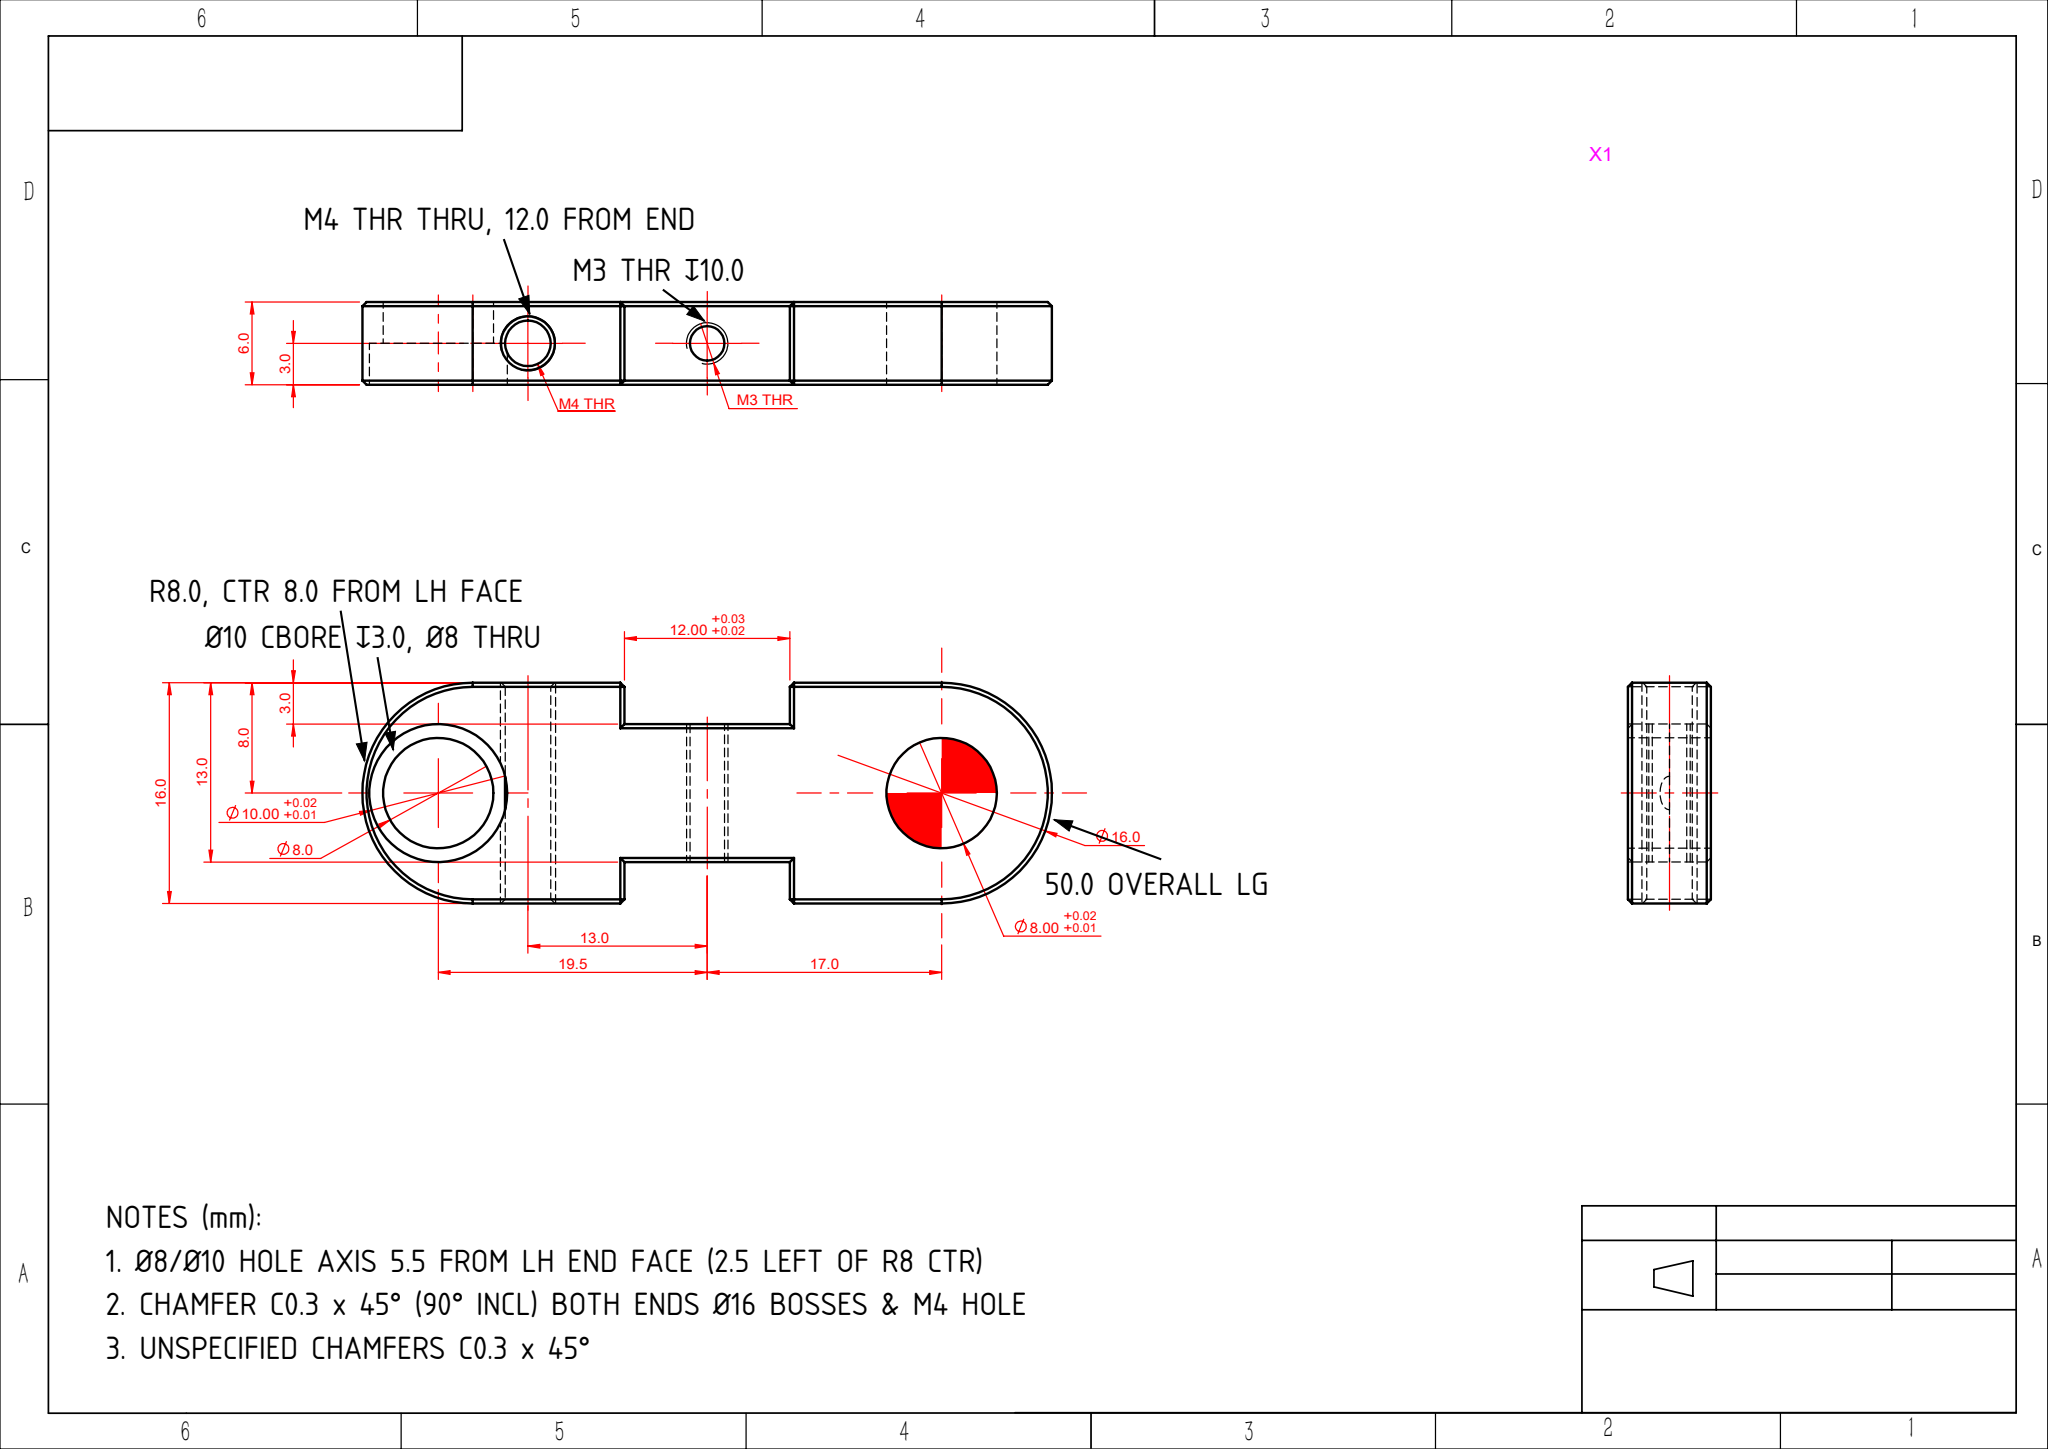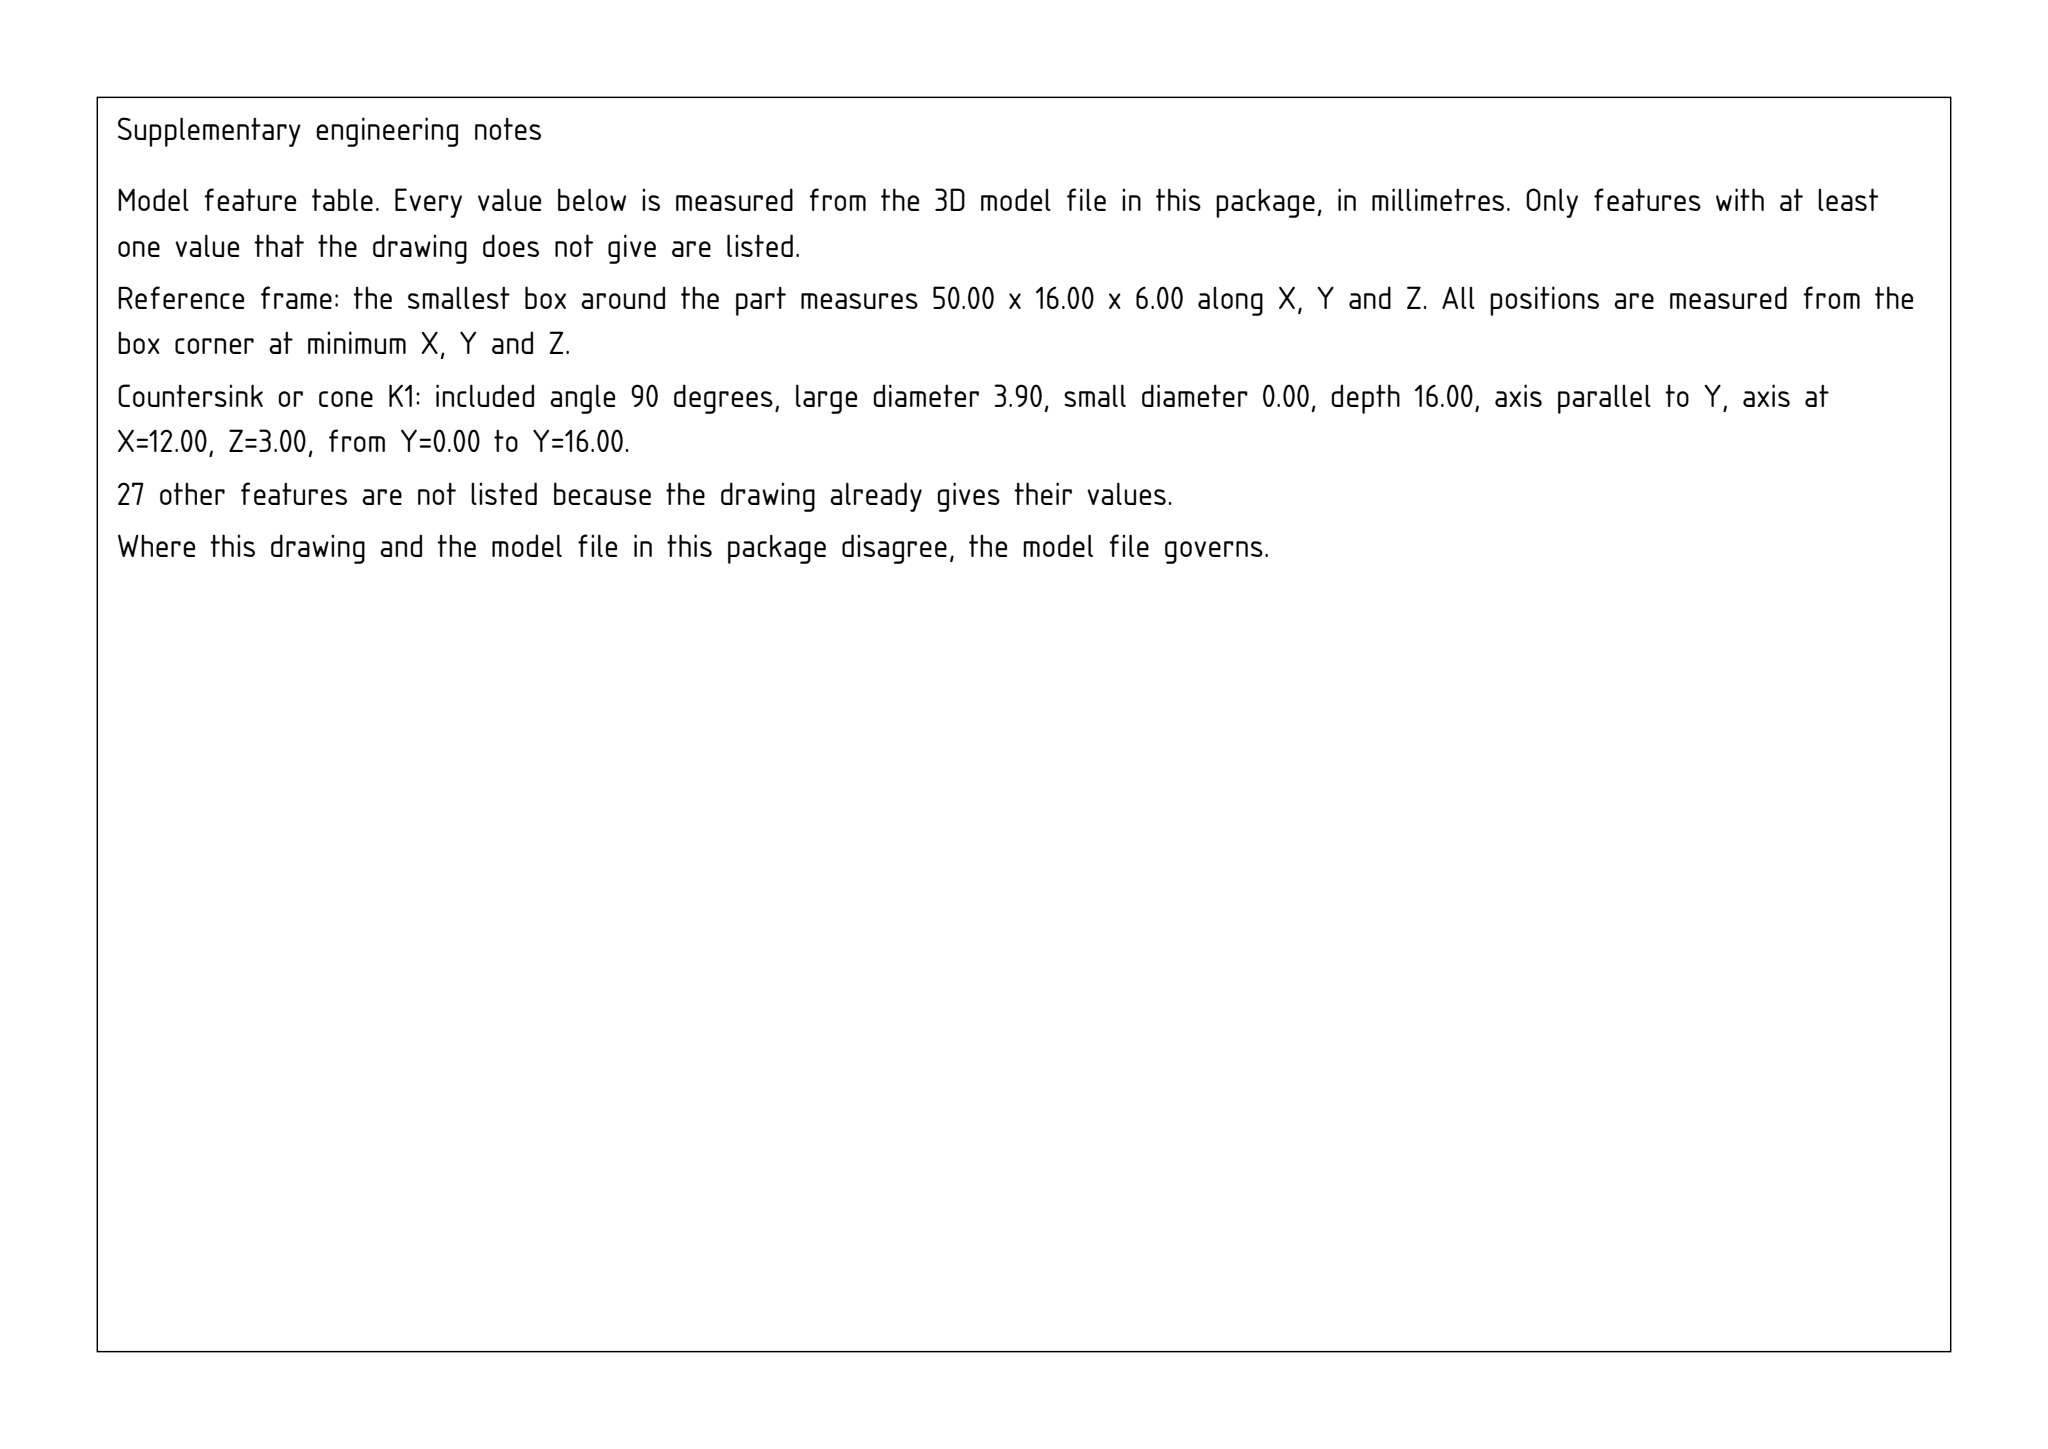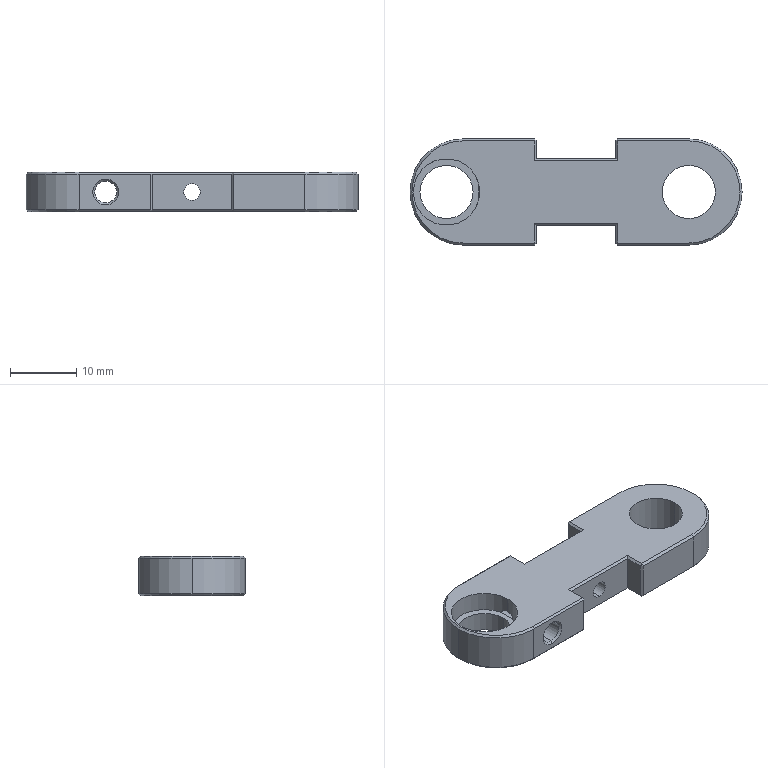Part | SolidWorks | mm | 1 solid | 68 faces | box 50 x 16 x 6 mm | volume 3151 mm3 | plane 45 | cylinder 13 | cone 10 | commonest cylinder face diameters 8 x4 16 x3 3.3 x2 2.5 x2 10 x2
Drawing notes:
OVERALL LG 50.0 | from the solid: bbox_xyz X = 50.0
Ø8/Ø10 HOLE AXIS 5.5 FROM LH END FACE (2.5 LEFT OF R8 CTR) | from the solid: Ø8 & Ø10 cyls at x=5.5; Ø16 LH arc ctr at x=8.0
Ø10.00 C'BORE DP 3.0, THEN Ø8.0 THRU (3.0 REMAINING) | from the solid: Ø10 z-cyl len 3.0 + Ø8 z-cyl len 3.0 at x=5.5; plate thk 6.0; z plane at 3.0
LH END R8.0 (Ø16.0), CTR 8.0 FROM LH END FACE | from the solid: Ø16 z-cyl at pos x=8.0, y=8.0
M3 THR DP 10.0 BLIND, AXIS 25.0 FROM LH END FACE | from the solid: Ø2.5 y-axis cyl at x=25.0, z=3.0, len 10.0 (part width 16.0)
M4 THR THRU, AXIS 12.0 FROM LH END FACE | from the solid: Ø3.3 y-axis cyl at x=12.0, z=3.0, len 15.4 + 0.3 chamf ea end = 16.0 width
CHAMFER C0.3 x 45° (90° INCL) BOTH ENDS Ø16 BOSSES & M4 HOLE | from the solid: cones 90° ref Ø16.0/15.4 and 90° ref Ø3.9/3.3 = 0.3 radial
UNSPECIFIED CHAMFERS C0.3 x 45° | from the solid: all cones 90° incl, 0.3 radial (Ø16→15.4, Ø3.9→3.3)
build123d program:
from build123d import *

# Parameters (mm, degrees)
BOSS_EXTRUDE1_DEPTH      = 6
F_8_0_8_DIAMETER_HOLE1_D = 8
SKETCH15_R               = 5
CUT_EXTRUDE5_DEPTH       = 3
SKETCH16_R               = 4
CUT_EXTRUDE6_DEPTH       = 27.42
SKETCH17_W               = 12
SKETCH17_H               = 6
CUT_EXTRUDE7_DEPTH       = 3
M3_TAPPED_HOLE2_D        = 2.5
M4_TAPPED_HOLE1_D        = 3.3
CHAMFER2_SIZE            = 0.3


with BuildPart() as part:
    # Sketch12 → Boss-Extrude1 (new body)
    with BuildSketch(Plane.XY):
        with BuildLine():
            Line((17, -8), (-17, -8))
            ThreePointArc((-17, -8), (-25, 0), (-17, 8))
            Line((-17, 8), (17, 8))
            ThreePointArc((17, 8), (25, 0), (17, -8))
        make_face()
    extrude(amount=BOSS_EXTRUDE1_DEPTH)

    # 8.0 _8_ Diameter Hole1 (through all)
    with Locations(Plane.XY.offset(6)):
        with Locations((17, 0)):
            Hole(F_8_0_8_DIAMETER_HOLE1_D / 2)

    # Sketch15 → Cut-Extrude5 (cut)
    with BuildSketch(Plane.XY.offset(6)):
        with Locations((-19.5, 0)):
            Circle(SKETCH15_R)
    extrude(amount=-CUT_EXTRUDE5_DEPTH, mode=Mode.SUBTRACT)

    # Sketch16 → Cut-Extrude6 (cut, through all)
    with BuildSketch(Plane.XY.offset(3)):
        with Locations((-19.5, 0)):
            Circle(SKETCH16_R)
    extrude(amount=-CUT_EXTRUDE6_DEPTH, mode=Mode.SUBTRACT)

    # Sketch17 → Cut-Extrude7 (cut)
    with BuildSketch(Plane(origin=(0, 8, 0), x_dir=(1, 0, 0), z_dir=(0, 1, 0))):
        with Locations((0, -3)):
            Rectangle(SKETCH17_W, SKETCH17_H)
    cut_extrude7 = extrude(amount=-CUT_EXTRUDE7_DEPTH, mode=Mode.SUBTRACT)

    # M3 Tapped Hole2 (through all)
    with Locations(Plane(origin=(0, 5, 0), x_dir=(1, 0, 0), z_dir=(0, 1, 0))):
        with Locations((0, -3)):
            Hole(M3_TAPPED_HOLE2_D / 2)

    # Mirror1: Cut-Extrude7 across plane
    add(cut_extrude7.mirror(Plane.ZX), mode=Mode.SUBTRACT)

    # M4 Tapped Hole1 (through all)
    with Locations(Plane(origin=(0, -8, 0), x_dir=(-1, 0, 0), z_dir=(0, -1, 0))):
        with Locations((13, -3)):
            Hole(M4_TAPPED_HOLE1_D / 2)

    # Chamfer2
    chamfer2_edges = [part.edges().sort_by_distance(p)[0] for p in [
        (-25, 0, 6),
        (-11.5, -8, 6),
        (-11.5, 8, 0),
        (-11.5, 8, 6),
        (6, 6.5, 0),
        (0, 5, 6),
        (6, 6.5, 6),
        (-6, 6.5, 6),
        (0, 5, 0),
        (-6, 6.5, 0),
        (6, 8, 3),
        (-6, 8, 3),
        (25, 0, 6),
        (-11.5, -8, 0),
        (11.5, -8, 0),
        (-25, 0, 0),
        (11.5, -8, 6),
        (11.5, 8, 0),
        (0, -5, 0),
        (0, -5, 6),
        (6, -8, 3),
        (6, -6.5, 6),
        (6, -6.5, 0),
        (-6, -8, 3),
        (-6, -6.5, 0),
        (-6, -6.5, 6),
        (25, 0, 0),
        (-14.65, -8, 3),
        (-14.65, 8, 3),
        (11.5, 8, 6),
    ]]
    chamfer(chamfer2_edges, length=CHAMFER2_SIZE)


solid = part.part